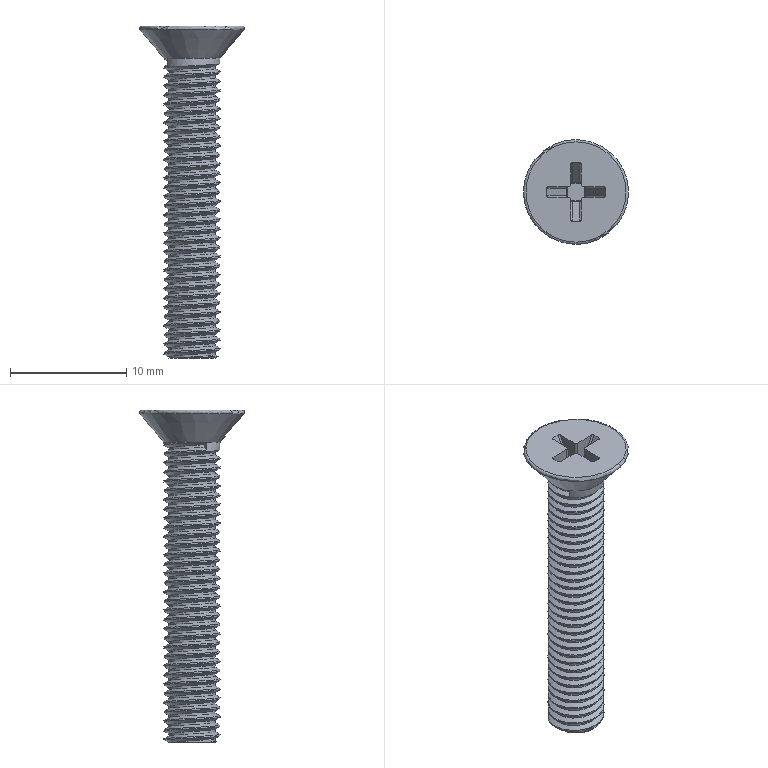Component | NX | MOUNTINGSCREW_3 | 1 solid | 40 faces | volume 489 mm3 | cylinder 18 | plane 16 | spline 3 | cone 2 | torus 1 | commonest cylinder face diameters 0.26 x12 0.4 x4 4.826 x1 4.032 x1